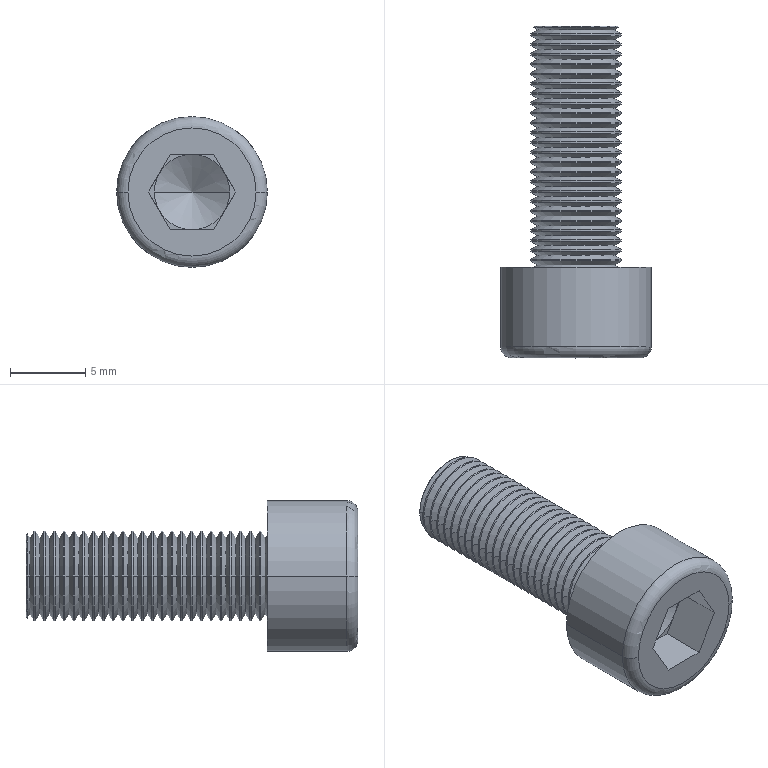Component | SolidWorks | LongSideClampingAssemblyBGeneralAssembly-1_HexSocketHeadCap-M6X16-0510-2 | 1 solid | 174 faces | box 10 x 22 x 10 mm | volume 787 mm3 | cone 104 | cylinder 52 | plane 16 | torus 2 | commonest cylinder face diameters 6 x48 10 x2 7.083 x2
build123d program:
from build123d import *

# Parameters (mm, degrees)
SKETCH1_R           = 5
BASEHEAD_DEPTH      = 6
SKETCH2_R           = 3
BASEBODY_DEPTH      = 16
HEXAGONSOCKET_DEPTH = 3
TOPFILLET_R         = 0.75
CHAMFER1_SIZE       = 0.25
LPATTERN10_COUNT    = 25
LPATTERN10_PITCH    = 0.6498


with BuildPart() as part:
    # Sketch1 → BaseHead (new body)
    with BuildSketch(Plane(origin=(0, 0, 0), x_dir=(0, 0, -1), z_dir=(1, 0, 0))):
        Circle(SKETCH1_R)
    extrude(amount=BASEHEAD_DEPTH)

    # Sketch2 → BaseBody (add)
    with BuildSketch(Plane(origin=(6, 0, 0), x_dir=(0, 0, -1), z_dir=(1, 0, 0))):
        Circle(SKETCH2_R)
    extrude(amount=BASEBODY_DEPTH)

    # Sketch3 → HexagonSocket (cut)
    with BuildSketch(Plane(origin=(0, 0, 0), x_dir=(0, 0, -1), z_dir=(1, 0, 0))):
        Polygon((2.887, 0), (1.443, 2.5), (-1.443, 2.5), (-2.887, 0), (-1.443, -2.5), (1.443, -2.5), align=None)
    extrude(amount=HEXAGONSOCKET_DEPTH, mode=Mode.SUBTRACT)

    # Sketch4 → Cut-Revolve1 (revolve, cut)
    with BuildSketch(Plane(origin=(-4.196, 0.75, 0), x_dir=(-1, 0, 0), z_dir=(0, 0, 1)), mode=Mode.PRIVATE) as cut_revolve1_sk:
        Polygon((-7.196, 3.25), (-8.64, 0.75), (-7.196, 0.75), align=None)
    revolve(cut_revolve1_sk.sketch.rotate(Axis((0.839, 0, 0), (-1, 0, 0)), 90), axis=Axis((0.839, 0, 0), (-1, 0, 0)), mode=Mode.SUBTRACT)

    # TopFillet
    topfillet_edges = [part.edges().sort_by_distance(p)[0] for p in [
        (0, 0, 5),
    ]]
    fillet(topfillet_edges, radius=TOPFILLET_R)

    # Chamfer1
    chamfer1_edges = [part.edges().sort_by_distance(p)[0] for p in [
        (22, 0, 3),
    ]]
    chamfer(chamfer1_edges, length=CHAMFER1_SIZE)

    # Sketch5 → Cut-Revolve10 (revolve, cut)
    with BuildSketch(Plane.XY, mode=Mode.PRIVATE) as cut_revolve10_sk:
        Polygon((21.75, 2.531), (22.021, 3), (22.021, 3.542), (21.479, 3.542), (21.479, 3), align=None)
    cut_revolve10 = revolve(cut_revolve10_sk.sketch.rotate(Axis((0, 0, 0), (1, 0, 0)), 90), axis=Axis((0, 0, 0), (1, 0, 0)), mode=Mode.SUBTRACT)

    # LPattern10: Cut-Revolve10 ×25
    with Locations(*[(-i * LPATTERN10_PITCH, 0, 0) for i in range(1, LPATTERN10_COUNT)]):
        add(cut_revolve10, mode=Mode.SUBTRACT)


solid = part.part

# Placed as in the assembly
solid = solid.moved(Location((-3159.658, -141.809, 3531.5), (90, 90, 0)))